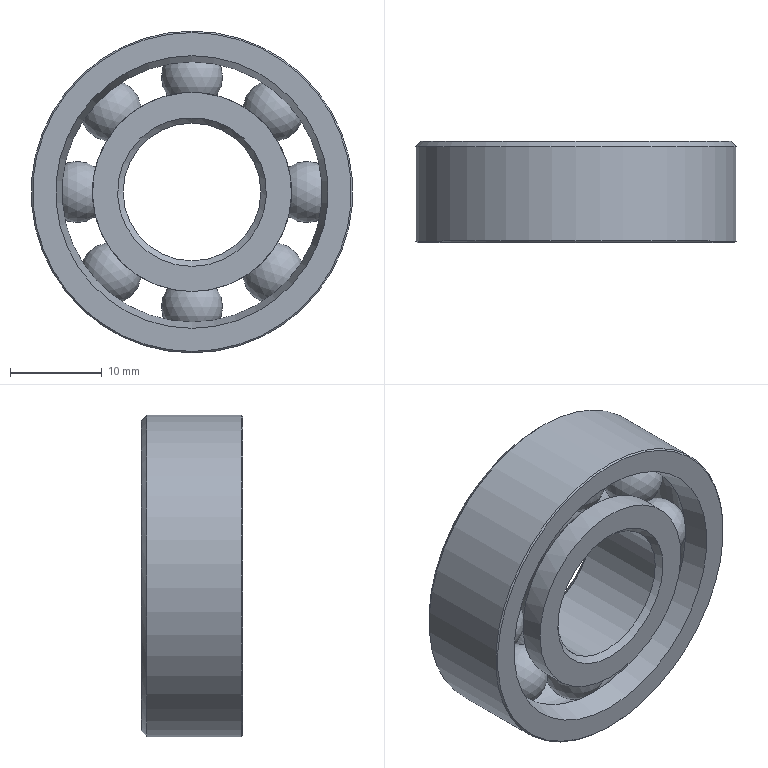Component | NX | GB-T292_AC-1994_7202_AC | 10 solids | 24 faces | volume 5812 mm3 | sphere 8 | cylinder 5 | cone 5 | plane 4 | torus 2 | commonest cylinder face diameters 21.667 x2 35 x1 28.333 x1 15 x1